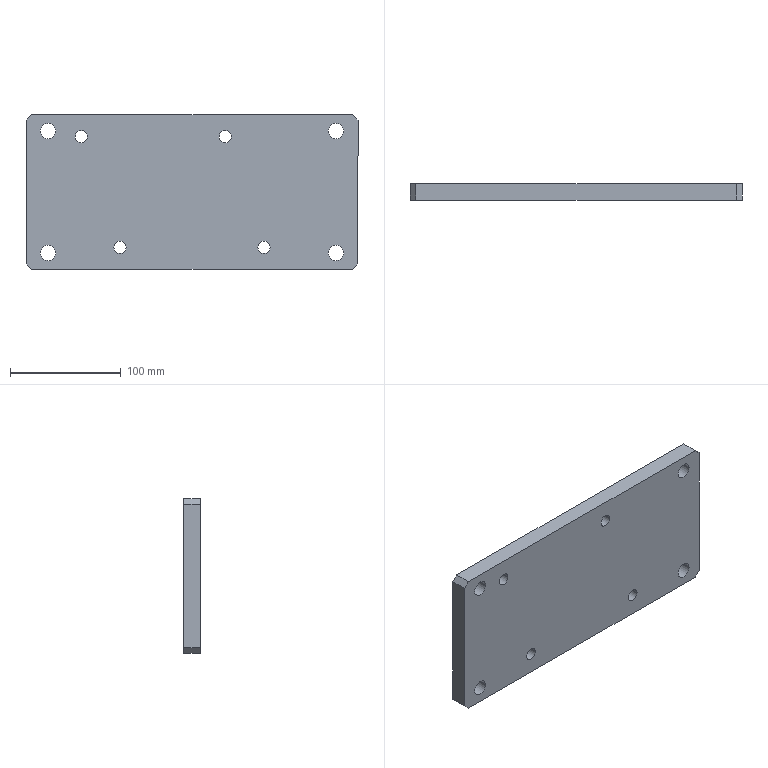Component | SolidWorks | LowerAdjustmentFrameBasePlate9.26-1 | 1 solid | 26 faces | box 300 x 15 x 140 mm | volume 614312 mm3 | cylinder 16 | plane 10 | commonest cylinder face diameters 11 x8 14 x8 | material AISI 1045 Steel, Cold Drawn
build123d program:
from build123d import *

# Parameters (mm, degrees)
SKETCH1_W           = 300
SKETCH1_H           = 140
BOSS_EXTRUDE1_DEPTH = 15
M14_TAPPED_HOLE1_D  = 14
CHAMFER1_SIZE       = 5
SKETCH4_R           = 5.5
CUT_EXTRUDE1_DEPTH  = 332.399


with BuildPart() as part:
    # Sketch1 → Boss-Extrude1 (new body)
    with BuildSketch(Plane.XY):
        with Locations((150, -70)):
            Rectangle(SKETCH1_W, SKETCH1_H)
    extrude(amount=BOSS_EXTRUDE1_DEPTH)

    # M14 Tapped Hole1 (through all)
    with Locations(Plane.XY.offset(15)):
        with Locations((20, -15), (280, -15), (280, -125), (20, -125)):
            Hole(M14_TAPPED_HOLE1_D / 2)

    # Chamfer1
    chamfer1_edges = [part.edges().sort_by_distance(p)[0] for p in [
        (0, 0, 7.5),
        (300, 0, 7.5),
        (300, -140, 7.5),
        (0, -140, 7.5),
    ]]
    chamfer(chamfer1_edges, length=CHAMFER1_SIZE)

    # Sketch4 → Cut-Extrude1 (cut, through all)
    with BuildSketch(Plane.XY.offset(15)):
        with Locations((215, -20)):
            Circle(SKETCH4_R)
        with Locations(Location((85, -20, 0), (0, 0, 180))):
            Circle(SKETCH4_R)
        with Locations((180, -120)):
            Circle(SKETCH4_R)
        with Locations((50, -120)):
            Circle(SKETCH4_R)
    extrude(amount=-CUT_EXTRUDE1_DEPTH, mode=Mode.SUBTRACT)


solid = part.part

# Placed as in the assembly
solid = solid.moved(Location((13.705, -428, -54.75), (-90, 0, 0)))